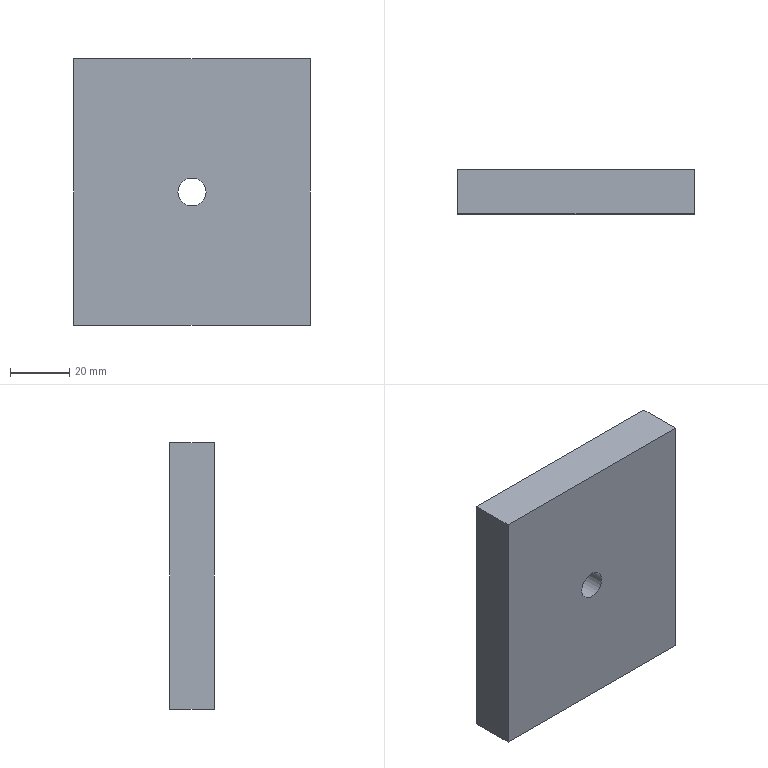Component | NX | CH3404_5-14 | 1 solid | 7 faces | box 80 x 15 x 90 mm | volume 106937 mm3 | plane 6 | cylinder 1 | commonest cylinder face diameters 9.5 x1
STEP:
#1=CARTESIAN_POINT('',(0.,0.,0.));
#2=DIRECTION('',(0.,0.,1.));
#3=DIRECTION('',(1.,0.,0.));
#4=AXIS2_PLACEMENT_3D('',#1,#2,#3);
#5=CARTESIAN_POINT('',(-275.,172.5,875.));
#6=VERTEX_POINT('',#5);
#7=CARTESIAN_POINT('',(-355.,172.5,875.));
#8=VERTEX_POINT('',#7);
#9=CARTESIAN_POINT('',(-275.,172.5,875.));
#10=DIRECTION('',(-1.,0.,0.));
#11=VECTOR('',#10,1.);
#12=LINE('',#9,#11);
#13=CARTESIAN_POINT('',(-275.,187.5,875.));
#14=DIRECTION('',(0.,0.,1.));
#15=DIRECTION('',(1.,0.,0.));
#16=AXIS2_PLACEMENT_3D('',#13,#14,#15);
#17=PLANE('',#16);
#18=CARTESIAN_POINT('',(0.,-15.));
#19=DIRECTION('',(-1.,0.));
#20=VECTOR('',#19,1.);
#21=LINE('',#18,#20);
#22=(GEOMETRIC_REPRESENTATION_CONTEXT(2)PARAMETRIC_REPRESENTATION_CONTEXT()REPRESENTATION_CONTEXT('',''));
#23=DEFINITIONAL_REPRESENTATION('',(#21),#22);
#24=PCURVE('',#17,#23);
#25=CARTESIAN_POINT('',(-315.,172.5,920.));
#26=DIRECTION('',(0.,1.,0.));
#27=DIRECTION('',(-1.,0.,0.));
#28=AXIS2_PLACEMENT_3D('',#25,#26,#27);
#29=PLANE('',#28);
#30=CARTESIAN_POINT('',(-40.,-45.));
#31=DIRECTION('',(1.,0.));
#32=VECTOR('',#31,1.);
#33=LINE('',#30,#32);
#34=(GEOMETRIC_REPRESENTATION_CONTEXT(2)PARAMETRIC_REPRESENTATION_CONTEXT()REPRESENTATION_CONTEXT('',''));
#35=DEFINITIONAL_REPRESENTATION('',(#33),#34);
#36=PCURVE('',#29,#35);
#37=SURFACE_CURVE('',#12,(#24,#36),.PCURVE_S1.);
#38=EDGE_CURVE('',#6,#8,#37,.T.);
#39=ORIENTED_EDGE('',*,*,#38,.T.);
#40=CARTESIAN_POINT('',(-355.,187.5,875.));
#41=VERTEX_POINT('',#40);
#42=CARTESIAN_POINT('',(-355.,187.5,875.));
#43=DIRECTION('',(0.,-1.,0.));
#44=VECTOR('',#43,1.);
#45=LINE('',#42,#44);
#46=CARTESIAN_POINT('',(-80.,0.));
#47=DIRECTION('',(0.,-1.));
#48=VECTOR('',#47,1.);
#49=LINE('',#46,#48);
#50=(GEOMETRIC_REPRESENTATION_CONTEXT(2)PARAMETRIC_REPRESENTATION_CONTEXT()REPRESENTATION_CONTEXT('',''));
#51=DEFINITIONAL_REPRESENTATION('',(#49),#50);
#52=PCURVE('',#17,#51);
#53=CARTESIAN_POINT('',(-355.,187.5,875.));
#54=DIRECTION('',(1.,0.,0.));
#55=DIRECTION('',(0.,1.,0.));
#56=AXIS2_PLACEMENT_3D('',#53,#54,#55);
#57=PLANE('',#56);
#58=CARTESIAN_POINT('',(0.,0.));
#59=DIRECTION('',(-1.,0.));
#60=VECTOR('',#59,1.);
#61=LINE('',#58,#60);
#62=(GEOMETRIC_REPRESENTATION_CONTEXT(2)PARAMETRIC_REPRESENTATION_CONTEXT()REPRESENTATION_CONTEXT('',''));
#63=DEFINITIONAL_REPRESENTATION('',(#61),#62);
#64=PCURVE('',#57,#63);
#65=SURFACE_CURVE('',#45,(#52,#64),.PCURVE_S1.);
#66=EDGE_CURVE('',#41,#8,#65,.T.);
#67=ORIENTED_EDGE('',*,*,#66,.F.);
#68=CARTESIAN_POINT('',(-275.,187.5,875.));
#69=VERTEX_POINT('',#68);
#70=CARTESIAN_POINT('',(-275.,187.5,875.));
#71=DIRECTION('',(-1.,0.,0.));
#72=VECTOR('',#71,1.);
#73=LINE('',#70,#72);
#74=CARTESIAN_POINT('',(0.,0.));
#75=DIRECTION('',(-1.,0.));
#76=VECTOR('',#75,1.);
#77=LINE('',#74,#76);
#78=(GEOMETRIC_REPRESENTATION_CONTEXT(2)PARAMETRIC_REPRESENTATION_CONTEXT()REPRESENTATION_CONTEXT('',''));
#79=DEFINITIONAL_REPRESENTATION('',(#77),#78);
#80=PCURVE('',#17,#79);
#81=CARTESIAN_POINT('',(-315.,187.5,920.));
#82=DIRECTION('',(0.,1.,0.));
#83=DIRECTION('',(-1.,0.,0.));
#84=AXIS2_PLACEMENT_3D('',#81,#82,#83);
#85=PLANE('',#84);
#86=CARTESIAN_POINT('',(-40.,-45.));
#87=DIRECTION('',(1.,0.));
#88=VECTOR('',#87,1.);
#89=LINE('',#86,#88);
#90=(GEOMETRIC_REPRESENTATION_CONTEXT(2)PARAMETRIC_REPRESENTATION_CONTEXT()REPRESENTATION_CONTEXT('',''));
#91=DEFINITIONAL_REPRESENTATION('',(#89),#90);
#92=PCURVE('',#85,#91);
#93=SURFACE_CURVE('',#73,(#80,#92),.PCURVE_S1.);
#94=EDGE_CURVE('',#69,#41,#93,.T.);
#95=ORIENTED_EDGE('',*,*,#94,.F.);
#96=CARTESIAN_POINT('',(-275.,187.5,875.));
#97=DIRECTION('',(0.,-1.,0.));
#98=VECTOR('',#97,1.);
#99=LINE('',#96,#98);
#100=CARTESIAN_POINT('',(0.,0.));
#101=DIRECTION('',(0.,-1.));
#102=VECTOR('',#101,1.);
#103=LINE('',#100,#102);
#104=(GEOMETRIC_REPRESENTATION_CONTEXT(2)PARAMETRIC_REPRESENTATION_CONTEXT()REPRESENTATION_CONTEXT('',''));
#105=DEFINITIONAL_REPRESENTATION('',(#103),#104);
#106=PCURVE('',#17,#105);
#107=CARTESIAN_POINT('',(-275.,187.5,965.));
#108=DIRECTION('',(-1.,0.,0.));
#109=DIRECTION('',(0.,-1.,0.));
#110=AXIS2_PLACEMENT_3D('',#107,#108,#109);
#111=PLANE('',#110);
#112=CARTESIAN_POINT('',(0.,-90.));
#113=DIRECTION('',(1.,0.));
#114=VECTOR('',#113,1.);
#115=LINE('',#112,#114);
#116=(GEOMETRIC_REPRESENTATION_CONTEXT(2)PARAMETRIC_REPRESENTATION_CONTEXT()REPRESENTATION_CONTEXT('',''));
#117=DEFINITIONAL_REPRESENTATION('',(#115),#116);
#118=PCURVE('',#111,#117);
#119=SURFACE_CURVE('',#99,(#106,#118),.PCURVE_S1.);
#120=EDGE_CURVE('',#69,#6,#119,.T.);
#121=ORIENTED_EDGE('',*,*,#120,.T.);
#122=EDGE_LOOP('',(#39,#67,#95,#121));
#123=FACE_BOUND('',#122,.T.);
#124=ADVANCED_FACE('',(#123),#17,.F.);
#125=CARTESIAN_POINT('',(-355.,172.5,965.));
#126=VERTEX_POINT('',#125);
#127=CARTESIAN_POINT('',(-355.,172.5,875.));
#128=DIRECTION('',(0.,0.,1.));
#129=VECTOR('',#128,1.);
#130=LINE('',#127,#129);
#131=CARTESIAN_POINT('',(-15.,0.));
#132=DIRECTION('',(0.,1.));
#133=VECTOR('',#132,1.);
#134=LINE('',#131,#133);
#135=(GEOMETRIC_REPRESENTATION_CONTEXT(2)PARAMETRIC_REPRESENTATION_CONTEXT()REPRESENTATION_CONTEXT('',''));
#136=DEFINITIONAL_REPRESENTATION('',(#134),#135);
#137=PCURVE('',#57,#136);
#138=CARTESIAN_POINT('',(40.,-45.));
#139=DIRECTION('',(0.,1.));
#140=VECTOR('',#139,1.);
#141=LINE('',#138,#140);
#142=(GEOMETRIC_REPRESENTATION_CONTEXT(2)PARAMETRIC_REPRESENTATION_CONTEXT()REPRESENTATION_CONTEXT('',''));
#143=DEFINITIONAL_REPRESENTATION('',(#141),#142);
#144=PCURVE('',#29,#143);
#145=SURFACE_CURVE('',#130,(#137,#144),.PCURVE_S1.);
#146=EDGE_CURVE('',#8,#126,#145,.T.);
#147=ORIENTED_EDGE('',*,*,#146,.T.);
#148=CARTESIAN_POINT('',(-355.,187.5,965.));
#149=VERTEX_POINT('',#148);
#150=CARTESIAN_POINT('',(-355.,187.5,965.));
#151=DIRECTION('',(0.,-1.,0.));
#152=VECTOR('',#151,1.);
#153=LINE('',#150,#152);
#154=CARTESIAN_POINT('',(0.,90.));
#155=DIRECTION('',(-1.,0.));
#156=VECTOR('',#155,1.);
#157=LINE('',#154,#156);
#158=(GEOMETRIC_REPRESENTATION_CONTEXT(2)PARAMETRIC_REPRESENTATION_CONTEXT()REPRESENTATION_CONTEXT('',''));
#159=DEFINITIONAL_REPRESENTATION('',(#157),#158);
#160=PCURVE('',#57,#159);
#161=CARTESIAN_POINT('',(-355.,187.5,965.));
#162=DIRECTION('',(0.,0.,-1.));
#163=DIRECTION('',(-1.,0.,0.));
#164=AXIS2_PLACEMENT_3D('',#161,#162,#163);
#165=PLANE('',#164);
#166=CARTESIAN_POINT('',(0.,0.));
#167=DIRECTION('',(0.,-1.));
#168=VECTOR('',#167,1.);
#169=LINE('',#166,#168);
#170=(GEOMETRIC_REPRESENTATION_CONTEXT(2)PARAMETRIC_REPRESENTATION_CONTEXT()REPRESENTATION_CONTEXT('',''));
#171=DEFINITIONAL_REPRESENTATION('',(#169),#170);
#172=PCURVE('',#165,#171);
#173=SURFACE_CURVE('',#153,(#160,#172),.PCURVE_S1.);
#174=EDGE_CURVE('',#149,#126,#173,.T.);
#175=ORIENTED_EDGE('',*,*,#174,.F.);
#176=CARTESIAN_POINT('',(-355.,187.5,875.));
#177=DIRECTION('',(0.,0.,1.));
#178=VECTOR('',#177,1.);
#179=LINE('',#176,#178);
#180=CARTESIAN_POINT('',(0.,0.));
#181=DIRECTION('',(0.,1.));
#182=VECTOR('',#181,1.);
#183=LINE('',#180,#182);
#184=(GEOMETRIC_REPRESENTATION_CONTEXT(2)PARAMETRIC_REPRESENTATION_CONTEXT()REPRESENTATION_CONTEXT('',''));
#185=DEFINITIONAL_REPRESENTATION('',(#183),#184);
#186=PCURVE('',#57,#185);
#187=CARTESIAN_POINT('',(40.,-45.));
#188=DIRECTION('',(0.,1.));
#189=VECTOR('',#188,1.);
#190=LINE('',#187,#189);
#191=(GEOMETRIC_REPRESENTATION_CONTEXT(2)PARAMETRIC_REPRESENTATION_CONTEXT()REPRESENTATION_CONTEXT('',''));
#192=DEFINITIONAL_REPRESENTATION('',(#190),#191);
#193=PCURVE('',#85,#192);
#194=SURFACE_CURVE('',#179,(#186,#193),.PCURVE_S1.);
#195=EDGE_CURVE('',#41,#149,#194,.T.);
#196=ORIENTED_EDGE('',*,*,#195,.F.);
#197=ORIENTED_EDGE('',*,*,#66,.T.);
#198=EDGE_LOOP('',(#147,#175,#196,#197));
#199=FACE_BOUND('',#198,.T.);
#200=ADVANCED_FACE('',(#199),#57,.F.);
#201=CARTESIAN_POINT('',(-275.,172.5,965.));
#202=VERTEX_POINT('',#201);
#203=CARTESIAN_POINT('',(-355.,172.5,965.));
#204=DIRECTION('',(1.,0.,0.));
#205=VECTOR('',#204,1.);
#206=LINE('',#203,#205);
#207=CARTESIAN_POINT('',(0.,-15.));
#208=DIRECTION('',(-1.,0.));
#209=VECTOR('',#208,1.);
#210=LINE('',#207,#209);
#211=(GEOMETRIC_REPRESENTATION_CONTEXT(2)PARAMETRIC_REPRESENTATION_CONTEXT()REPRESENTATION_CONTEXT('',''));
#212=DEFINITIONAL_REPRESENTATION('',(#210),#211);
#213=PCURVE('',#165,#212);
#214=CARTESIAN_POINT('',(40.,45.));
#215=DIRECTION('',(-1.,0.));
#216=VECTOR('',#215,1.);
#217=LINE('',#214,#216);
#218=(GEOMETRIC_REPRESENTATION_CONTEXT(2)PARAMETRIC_REPRESENTATION_CONTEXT()REPRESENTATION_CONTEXT('',''));
#219=DEFINITIONAL_REPRESENTATION('',(#217),#218);
#220=PCURVE('',#29,#219);
#221=SURFACE_CURVE('',#206,(#213,#220),.PCURVE_S1.);
#222=EDGE_CURVE('',#126,#202,#221,.T.);
#223=ORIENTED_EDGE('',*,*,#222,.T.);
#224=CARTESIAN_POINT('',(-275.,187.5,965.));
#225=VERTEX_POINT('',#224);
#226=CARTESIAN_POINT('',(-275.,187.5,965.));
#227=DIRECTION('',(0.,-1.,0.));
#228=VECTOR('',#227,1.);
#229=LINE('',#226,#228);
#230=CARTESIAN_POINT('',(-80.,0.));
#231=DIRECTION('',(0.,-1.));
#232=VECTOR('',#231,1.);
#233=LINE('',#230,#232);
#234=(GEOMETRIC_REPRESENTATION_CONTEXT(2)PARAMETRIC_REPRESENTATION_CONTEXT()REPRESENTATION_CONTEXT('',''));
#235=DEFINITIONAL_REPRESENTATION('',(#233),#234);
#236=PCURVE('',#165,#235);
#237=CARTESIAN_POINT('',(0.,0.));
#238=DIRECTION('',(1.,0.));
#239=VECTOR('',#238,1.);
#240=LINE('',#237,#239);
#241=(GEOMETRIC_REPRESENTATION_CONTEXT(2)PARAMETRIC_REPRESENTATION_CONTEXT()REPRESENTATION_CONTEXT('',''));
#242=DEFINITIONAL_REPRESENTATION('',(#240),#241);
#243=PCURVE('',#111,#242);
#244=SURFACE_CURVE('',#229,(#236,#243),.PCURVE_S1.);
#245=EDGE_CURVE('',#225,#202,#244,.T.);
#246=ORIENTED_EDGE('',*,*,#245,.F.);
#247=CARTESIAN_POINT('',(-355.,187.5,965.));
#248=DIRECTION('',(1.,0.,0.));
#249=VECTOR('',#248,1.);
#250=LINE('',#247,#249);
#251=CARTESIAN_POINT('',(0.,0.));
#252=DIRECTION('',(-1.,0.));
#253=VECTOR('',#252,1.);
#254=LINE('',#251,#253);
#255=(GEOMETRIC_REPRESENTATION_CONTEXT(2)PARAMETRIC_REPRESENTATION_CONTEXT()REPRESENTATION_CONTEXT('',''));
#256=DEFINITIONAL_REPRESENTATION('',(#254),#255);
#257=PCURVE('',#165,#256);
#258=CARTESIAN_POINT('',(40.,45.));
#259=DIRECTION('',(-1.,0.));
#260=VECTOR('',#259,1.);
#261=LINE('',#258,#260);
#262=(GEOMETRIC_REPRESENTATION_CONTEXT(2)PARAMETRIC_REPRESENTATION_CONTEXT()REPRESENTATION_CONTEXT('',''));
#263=DEFINITIONAL_REPRESENTATION('',(#261),#262);
#264=PCURVE('',#85,#263);
#265=SURFACE_CURVE('',#250,(#257,#264),.PCURVE_S1.);
#266=EDGE_CURVE('',#149,#225,#265,.T.);
#267=ORIENTED_EDGE('',*,*,#266,.F.);
#268=ORIENTED_EDGE('',*,*,#174,.T.);
#269=EDGE_LOOP('',(#223,#246,#267,#268));
#270=FACE_BOUND('',#269,.T.);
#271=ADVANCED_FACE('',(#270),#165,.F.);
#272=CARTESIAN_POINT('',(-275.,172.5,965.));
#273=DIRECTION('',(0.,0.,-1.));
#274=VECTOR('',#273,1.);
#275=LINE('',#272,#274);
#276=CARTESIAN_POINT('',(15.,0.));
#277=DIRECTION('',(0.,-1.));
#278=VECTOR('',#277,1.);
#279=LINE('',#276,#278);
#280=(GEOMETRIC_REPRESENTATION_CONTEXT(2)PARAMETRIC_REPRESENTATION_CONTEXT()REPRESENTATION_CONTEXT('',''));
#281=DEFINITIONAL_REPRESENTATION('',(#279),#280);
#282=PCURVE('',#111,#281);
#283=CARTESIAN_POINT('',(-40.,45.));
#284=DIRECTION('',(0.,-1.));
#285=VECTOR('',#284,1.);
#286=LINE('',#283,#285);
#287=(GEOMETRIC_REPRESENTATION_CONTEXT(2)PARAMETRIC_REPRESENTATION_CONTEXT()REPRESENTATION_CONTEXT('',''));
#288=DEFINITIONAL_REPRESENTATION('',(#286),#287);
#289=PCURVE('',#29,#288);
#290=SURFACE_CURVE('',#275,(#282,#289),.PCURVE_S1.);
#291=EDGE_CURVE('',#202,#6,#290,.T.);
#292=ORIENTED_EDGE('',*,*,#291,.T.);
#293=ORIENTED_EDGE('',*,*,#120,.F.);
#294=CARTESIAN_POINT('',(-275.,187.5,965.));
#295=DIRECTION('',(0.,0.,-1.));
#296=VECTOR('',#295,1.);
#297=LINE('',#294,#296);
#298=CARTESIAN_POINT('',(0.,0.));
#299=DIRECTION('',(0.,-1.));
#300=VECTOR('',#299,1.);
#301=LINE('',#298,#300);
#302=(GEOMETRIC_REPRESENTATION_CONTEXT(2)PARAMETRIC_REPRESENTATION_CONTEXT()REPRESENTATION_CONTEXT('',''));
#303=DEFINITIONAL_REPRESENTATION('',(#301),#302);
#304=PCURVE('',#111,#303);
#305=CARTESIAN_POINT('',(-40.,45.));
#306=DIRECTION('',(0.,-1.));
#307=VECTOR('',#306,1.);
#308=LINE('',#305,#307);
#309=(GEOMETRIC_REPRESENTATION_CONTEXT(2)PARAMETRIC_REPRESENTATION_CONTEXT()REPRESENTATION_CONTEXT('',''));
#310=DEFINITIONAL_REPRESENTATION('',(#308),#309);
#311=PCURVE('',#85,#310);
#312=SURFACE_CURVE('',#297,(#304,#311),.PCURVE_S1.);
#313=EDGE_CURVE('',#225,#69,#312,.T.);
#314=ORIENTED_EDGE('',*,*,#313,.F.);
#315=ORIENTED_EDGE('',*,*,#245,.T.);
#316=EDGE_LOOP('',(#292,#293,#314,#315));
#317=FACE_BOUND('',#316,.T.);
#318=ADVANCED_FACE('',(#317),#111,.F.);
#319=CARTESIAN_POINT('',(-310.25,187.5,920.));
#320=VERTEX_POINT('',#319);
#321=CARTESIAN_POINT('',(-315.,187.5,920.));
#322=DIRECTION('',(0.,-1.,0.));
#323=DIRECTION('',(1.,0.,0.));
#324=AXIS2_PLACEMENT_3D('',#321,#322,#323);
#325=CIRCLE('',#324,4.75);
#326=CARTESIAN_POINT('',(-4.75,0.));
#327=CARTESIAN_POINT('',(-4.75,8.227));
#328=CARTESIAN_POINT('',(2.375,4.114));
#329=CARTESIAN_POINT('',(9.5,0.));
#330=CARTESIAN_POINT('',(2.375,-4.114));
#331=CARTESIAN_POINT('',(-4.75,-8.227));
#332=CARTESIAN_POINT('',(-4.75,0.));
#333=(BOUNDED_CURVE()B_SPLINE_CURVE(2,(#326,#327,#328,#329,#330,#331,#332),.UNSPECIFIED.,.T.,.F.)B_SPLINE_CURVE_WITH_KNOTS((1,2,2,2,2,1),(-2.094,0.,2.094,4.189,6.283,8.378),.UNSPECIFIED.)CURVE()GEOMETRIC_REPRESENTATION_ITEM()RATIONAL_B_SPLINE_CURVE((1.,0.5,1.,0.5,1.,0.5,1.))REPRESENTATION_ITEM(''));
#334=(GEOMETRIC_REPRESENTATION_CONTEXT(2)PARAMETRIC_REPRESENTATION_CONTEXT()REPRESENTATION_CONTEXT('',''));
#335=DEFINITIONAL_REPRESENTATION('',(#333),#334);
#336=PCURVE('',#85,#335);
#337=CARTESIAN_POINT('',(-315.,187.5,920.));
#338=DIRECTION('',(0.,-1.,0.));
#339=DIRECTION('',(1.,0.,0.));
#340=AXIS2_PLACEMENT_3D('',#337,#338,#339);
#341=CYLINDRICAL_SURFACE('',#340,4.75);
#342=CARTESIAN_POINT('',(0.,0.));
#343=DIRECTION('',(1.,0.));
#344=VECTOR('',#343,1.);
#345=LINE('',#342,#344);
#346=(GEOMETRIC_REPRESENTATION_CONTEXT(2)PARAMETRIC_REPRESENTATION_CONTEXT()REPRESENTATION_CONTEXT('',''));
#347=DEFINITIONAL_REPRESENTATION('',(#345),#346);
#348=PCURVE('',#341,#347);
#349=SURFACE_CURVE('',#325,(#336,#348),.PCURVE_S1.);
#350=EDGE_CURVE('',#320,#320,#349,.T.);
#351=ORIENTED_EDGE('',*,*,#350,.T.);
#352=EDGE_LOOP('',(#351));
#353=FACE_BOUND('',#352,.T.);
#354=ORIENTED_EDGE('',*,*,#94,.T.);
#355=ORIENTED_EDGE('',*,*,#195,.T.);
#356=ORIENTED_EDGE('',*,*,#266,.T.);
#357=ORIENTED_EDGE('',*,*,#313,.T.);
#358=EDGE_LOOP('',(#354,#355,#356,#357));
#359=FACE_BOUND('',#358,.T.);
#360=ADVANCED_FACE('',(#353,#359),#85,.T.);
#361=CARTESIAN_POINT('',(-319.75,172.5,920.));
#362=VERTEX_POINT('',#361);
#363=CARTESIAN_POINT('',(-310.25,172.5,920.));
#364=VERTEX_POINT('',#363);
#365=CARTESIAN_POINT('',(-315.,172.5,920.));
#366=DIRECTION('',(0.,1.,0.));
#367=DIRECTION('',(-1.,0.,0.));
#368=AXIS2_PLACEMENT_3D('',#365,#366,#367);
#369=CIRCLE('',#368,4.75);
#370=CARTESIAN_POINT('',(0.,0.));
#371=DIRECTION('',(1.,0.));
#372=AXIS2_PLACEMENT_2D('',#370,#371);
#373=CIRCLE('',#372,4.75);
#374=(GEOMETRIC_REPRESENTATION_CONTEXT(2)PARAMETRIC_REPRESENTATION_CONTEXT()REPRESENTATION_CONTEXT('',''));
#375=DEFINITIONAL_REPRESENTATION('',(#373),#374);
#376=PCURVE('',#29,#375);
#377=CARTESIAN_POINT('',(3.142,15.));
#378=DIRECTION('',(-1.,0.));
#379=VECTOR('',#378,1.);
#380=LINE('',#377,#379);
#381=(GEOMETRIC_REPRESENTATION_CONTEXT(2)PARAMETRIC_REPRESENTATION_CONTEXT()REPRESENTATION_CONTEXT('',''));
#382=DEFINITIONAL_REPRESENTATION('',(#380),#381);
#383=PCURVE('',#341,#382);
#384=SURFACE_CURVE('',#369,(#376,#383),.PCURVE_S1.);
#385=EDGE_CURVE('',#362,#364,#384,.T.);
#386=ORIENTED_EDGE('',*,*,#385,.T.);
#387=CARTESIAN_POINT('',(-315.,172.5,920.));
#388=DIRECTION('',(0.,1.,0.));
#389=DIRECTION('',(-1.,0.,0.));
#390=AXIS2_PLACEMENT_3D('',#387,#388,#389);
#391=CIRCLE('',#390,4.75);
#392=CARTESIAN_POINT('',(0.,0.));
#393=DIRECTION('',(1.,0.));
#394=AXIS2_PLACEMENT_2D('',#392,#393);
#395=CIRCLE('',#394,4.75);
#396=(GEOMETRIC_REPRESENTATION_CONTEXT(2)PARAMETRIC_REPRESENTATION_CONTEXT()REPRESENTATION_CONTEXT('',''));
#397=DEFINITIONAL_REPRESENTATION('',(#395),#396);
#398=PCURVE('',#29,#397);
#399=CARTESIAN_POINT('',(9.425,15.));
#400=DIRECTION('',(-1.,0.));
#401=VECTOR('',#400,1.);
#402=LINE('',#399,#401);
#403=(GEOMETRIC_REPRESENTATION_CONTEXT(2)PARAMETRIC_REPRESENTATION_CONTEXT()REPRESENTATION_CONTEXT('',''));
#404=DEFINITIONAL_REPRESENTATION('',(#402),#403);
#405=PCURVE('',#341,#404);
#406=SURFACE_CURVE('',#391,(#398,#405),.PCURVE_S1.);
#407=EDGE_CURVE('',#364,#362,#406,.T.);
#408=ORIENTED_EDGE('',*,*,#407,.T.);
#409=EDGE_LOOP('',(#386,#408));
#410=FACE_BOUND('',#409,.T.);
#411=ORIENTED_EDGE('',*,*,#38,.F.);
#412=ORIENTED_EDGE('',*,*,#291,.F.);
#413=ORIENTED_EDGE('',*,*,#222,.F.);
#414=ORIENTED_EDGE('',*,*,#146,.F.);
#415=EDGE_LOOP('',(#411,#412,#413,#414));
#416=FACE_BOUND('',#415,.T.);
#417=ADVANCED_FACE('',(#410,#416),#29,.F.);
#418=ORIENTED_EDGE('',*,*,#350,.T.);
#419=CARTESIAN_POINT('',(-310.25,187.5,920.));
#420=CARTESIAN_POINT('',(-310.25,172.5,920.));
#421=B_SPLINE_CURVE_WITH_KNOTS('',1,(#419,#420),.UNSPECIFIED.,.F.,.F.,(2,2),(0.,15.),.PIECEWISE_BEZIER_KNOTS.);
#422=CARTESIAN_POINT('',(6.283,0.));
#423=DIRECTION('',(0.,1.));
#424=VECTOR('',#423,1.);
#425=LINE('',#422,#424);
#426=(GEOMETRIC_REPRESENTATION_CONTEXT(2)PARAMETRIC_REPRESENTATION_CONTEXT()REPRESENTATION_CONTEXT('',''));
#427=DEFINITIONAL_REPRESENTATION('',(#425),#426);
#428=PCURVE('',#341,#427);
#429=CARTESIAN_POINT('',(0.,0.));
#430=DIRECTION('',(0.,1.));
#431=VECTOR('',#430,1.);
#432=LINE('',#429,#431);
#433=(GEOMETRIC_REPRESENTATION_CONTEXT(2)PARAMETRIC_REPRESENTATION_CONTEXT()REPRESENTATION_CONTEXT('',''));
#434=DEFINITIONAL_REPRESENTATION('',(#432),#433);
#435=PCURVE('',#341,#434);
#436=SEAM_CURVE('',#421,(#428,#435),.PCURVE_S1.);
#437=EDGE_CURVE('',#320,#364,#436,.T.);
#438=ORIENTED_EDGE('',*,*,#437,.T.);
#439=ORIENTED_EDGE('',*,*,#407,.T.);
#440=ORIENTED_EDGE('',*,*,#385,.T.);
#441=ORIENTED_EDGE('',*,*,#437,.F.);
#442=EDGE_LOOP('',(#418,#438,#439,#440,#441));
#443=FACE_BOUND('',#442,.F.);
#444=ADVANCED_FACE('',(#443),#341,.F.);
#445=CLOSED_SHELL('',(#124,#200,#271,#318,#360,#417,#444));
#446=MANIFOLD_SOLID_BREP('',#445);
#447=(LENGTH_UNIT()NAMED_UNIT(*)SI_UNIT(.MILLI.,.METRE.));
#448=UNCERTAINTY_MEASURE_WITH_UNIT(LENGTH_MEASURE(0.000002),#447,'','');
#449=(NAMED_UNIT(*)PLANE_ANGLE_UNIT()SI_UNIT($,.RADIAN.));
#450=(NAMED_UNIT(*)SI_UNIT($,.STERADIAN.)SOLID_ANGLE_UNIT());
#451=(GEOMETRIC_REPRESENTATION_CONTEXT(3)GLOBAL_UNCERTAINTY_ASSIGNED_CONTEXT((#448))GLOBAL_UNIT_ASSIGNED_CONTEXT((#447,#449,#450))REPRESENTATION_CONTEXT('',''));
#452=ADVANCED_BREP_SHAPE_REPRESENTATION('',(#4,#446),#451);